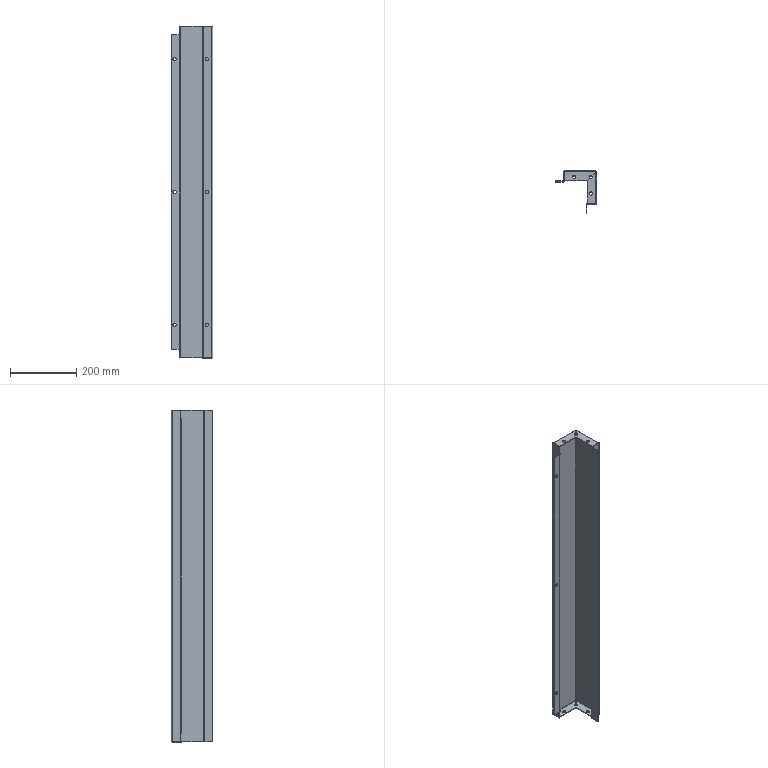Component | SolidWorks | 16UpperRightBeam-1 | 1 solid | 114 faces | volume 619049 mm3 | plane 66 | cylinder 44 | spline 4 | commonest cylinder face diameters 10 x26 6 x9 2 x9